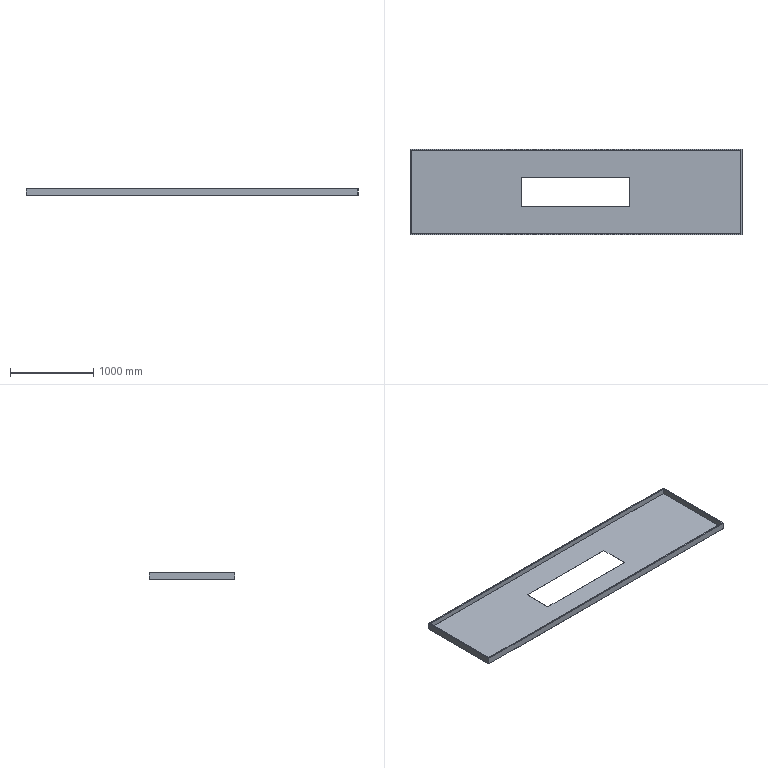Component | NX | DB10_12 | 1 solid | 20 faces | volume 6865527 mm3 | plane 20